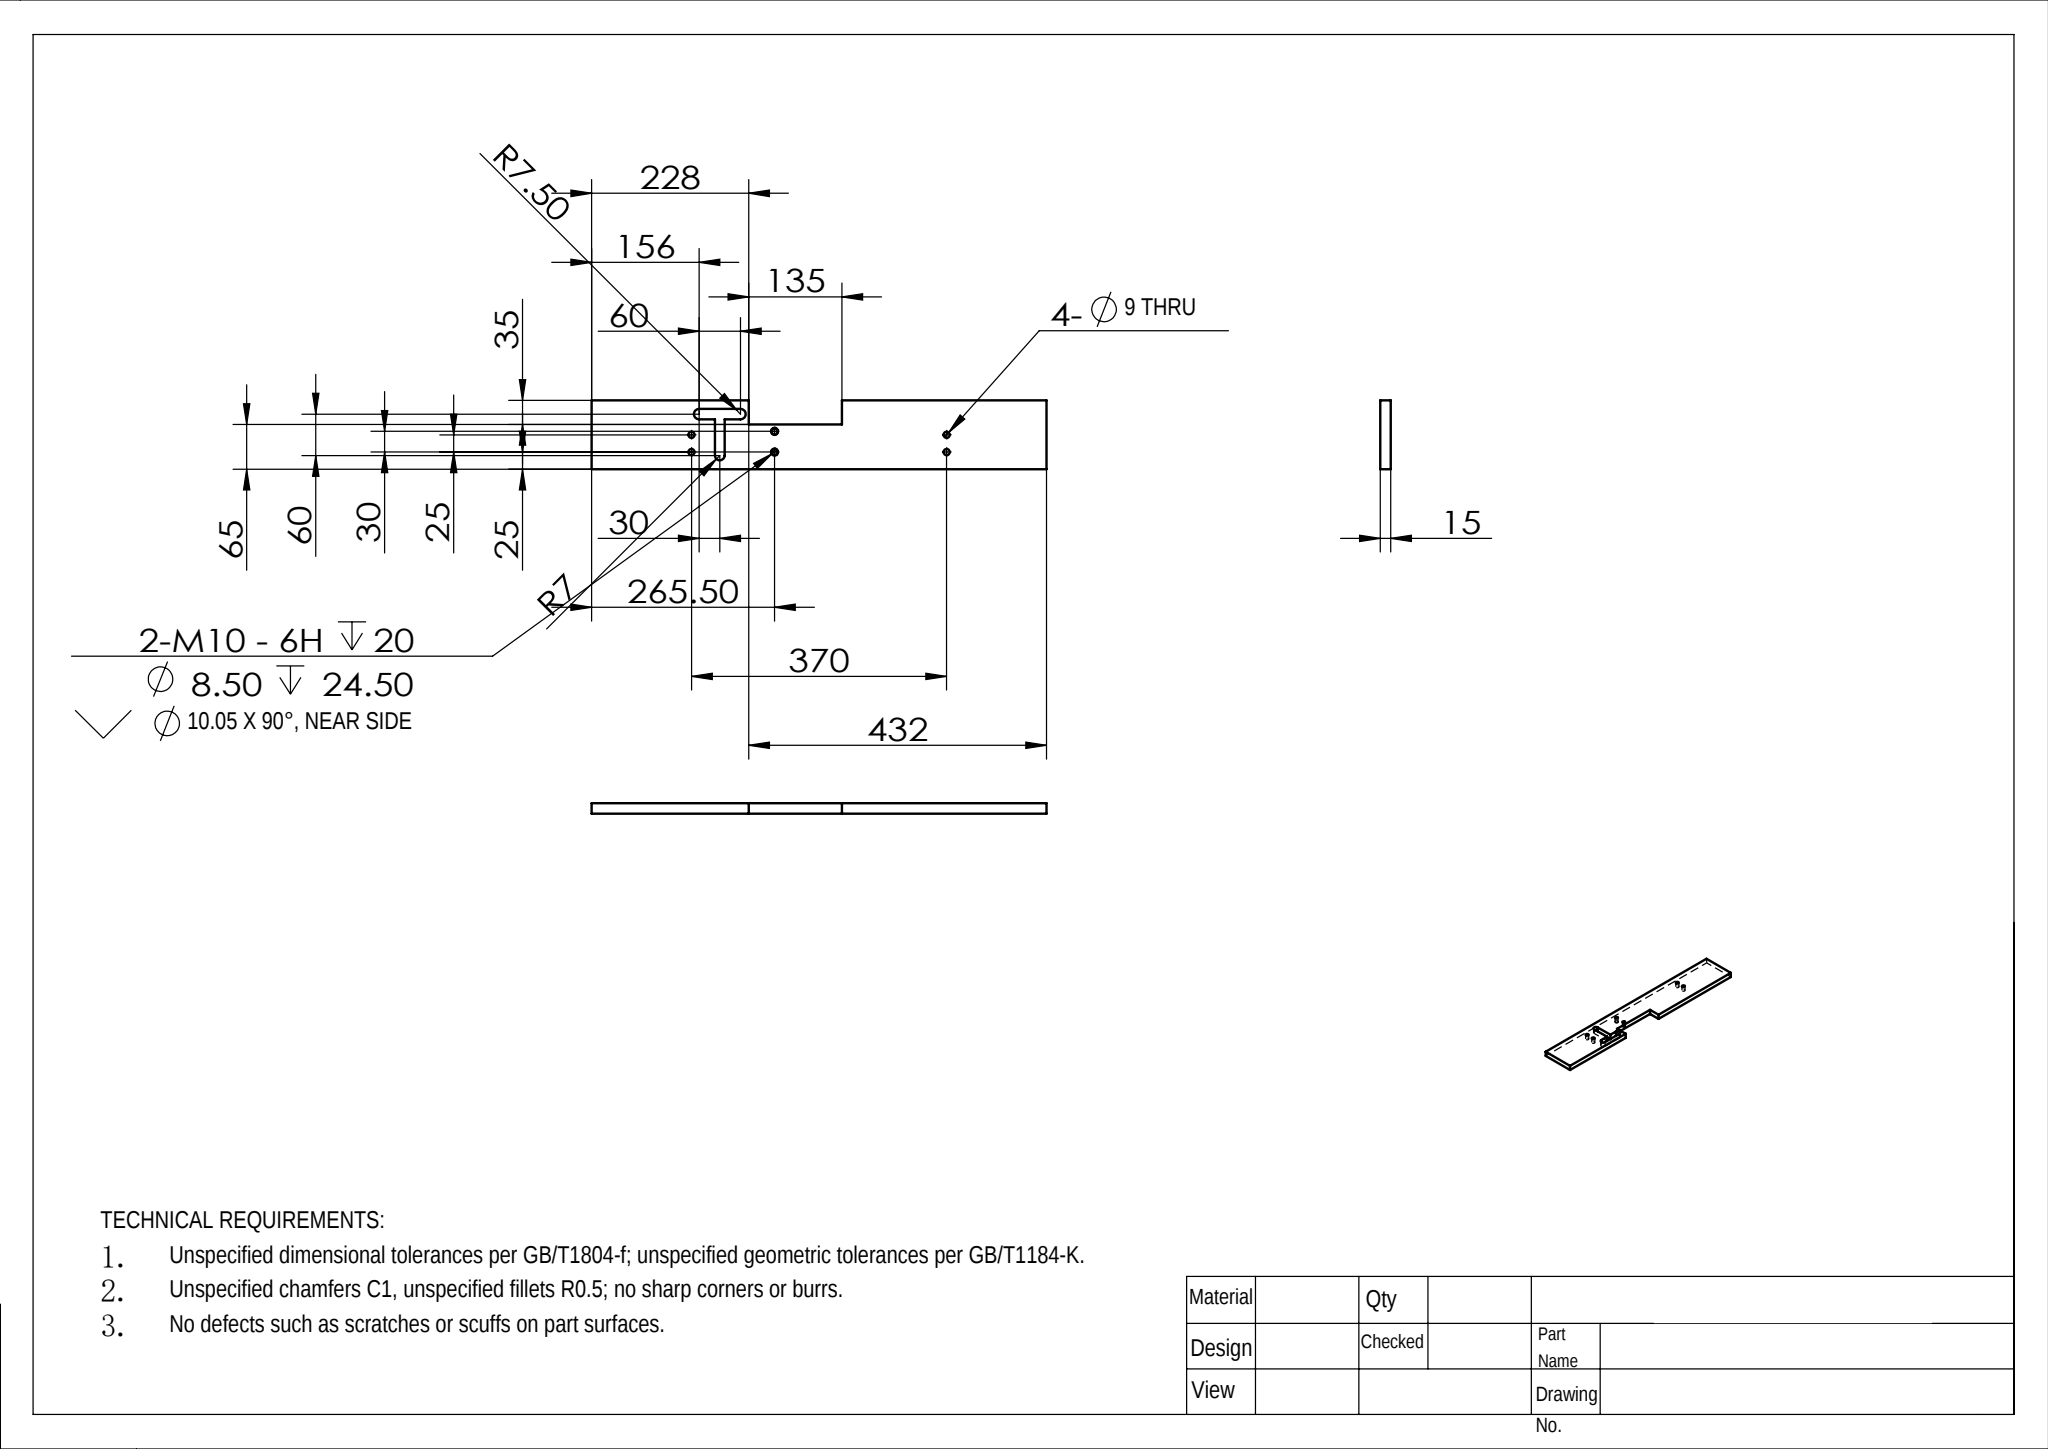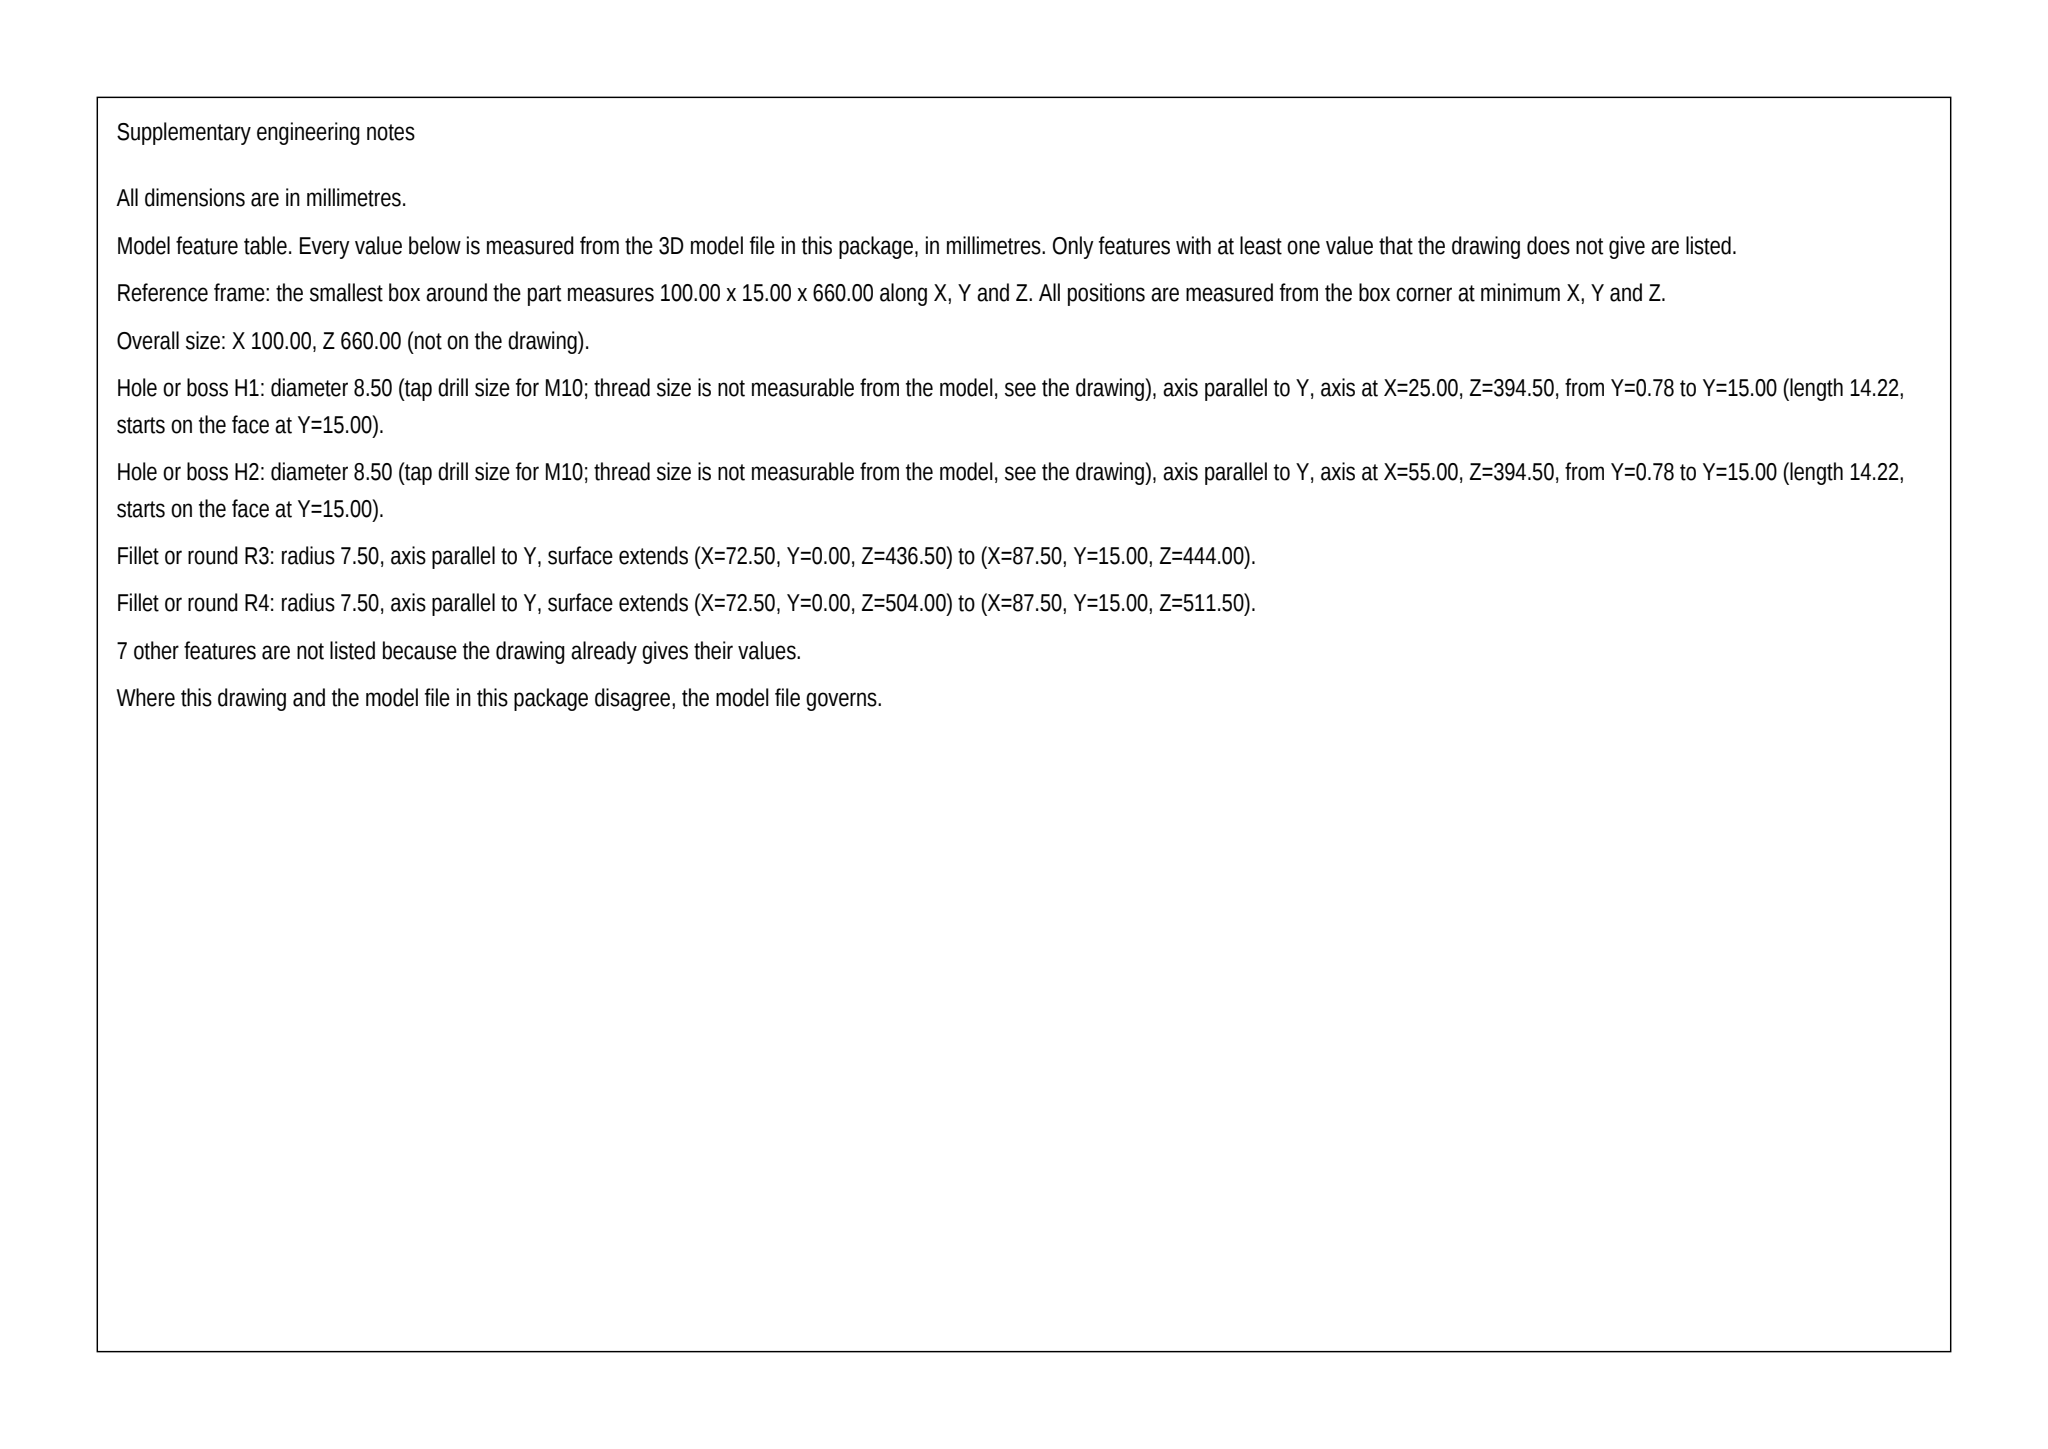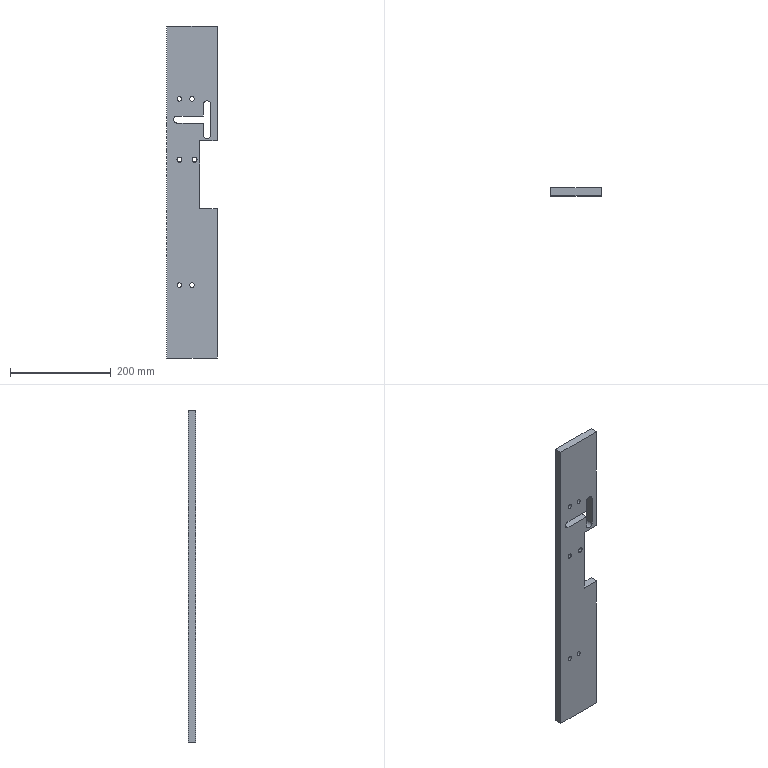Part | SolidWorks | mm | 1 solid | 35 faces | box 100 x 15 x 660 mm | volume 885258 mm3 | cylinder 16 | plane 15 | cone 4 | commonest cylinder face diameters 9 x8 8.5 x4 15 x3 14 x1
build123d program:
from build123d import *

# Parameters (mm, degrees)
SKETCH1_W                    = 100
SKETCH1_H                    = 660
BOSS_EXTRUDE1_DEPTH          = 15
M10_TAPPED_HOLE1_D           = 8.5
M10_TAPPED_HOLE1_DEPTH       = 24.5
M10_TAPPED_HOLE1_CSINK_D     = 10.05
M10_TAPPED_HOLE1_CSINK_ANGLE = 90
M10_TAPPED_HOLE1_TIP         = 2.554
SKETCH5_W                    = 66.431
SKETCH5_H                    = 135
CUT_EXTRUDE1_DEPTH           = 668.701
SKETCH6_R                    = 4.5
CUT_EXTRUDE2_DEPTH           = 668.701
CUT_EXTRUDE3_DEPTH           = 668.701
CUT_EXTRUDE4_DEPTH           = 668.701


with BuildPart() as part:
    # Sketch1 → Boss-Extrude1 (new body)
    with BuildSketch(Plane(origin=(0, 0, 0), x_dir=(1, 0, 0), z_dir=(0, 1, 0))):
        with Locations((50, 330)):
            Rectangle(SKETCH1_W, SKETCH1_H)
    extrude(amount=BOSS_EXTRUDE1_DEPTH)

    # M10 Tapped Hole1
    with Locations(Plane(origin=(0, 0, 0), x_dir=(-1, 0, 0), z_dir=(0, -1, 0))):
        with Locations((-55, 265.5), (-25, 265.5)):
            CounterSinkHole(M10_TAPPED_HOLE1_D / 2, M10_TAPPED_HOLE1_CSINK_D / 2, depth=M10_TAPPED_HOLE1_DEPTH, counter_sink_angle=M10_TAPPED_HOLE1_CSINK_ANGLE)
            with Locations((0, 0, -(M10_TAPPED_HOLE1_DEPTH + M10_TAPPED_HOLE1_TIP / 2))):  # 118° drill point
                Cone(0, M10_TAPPED_HOLE1_D / 2, M10_TAPPED_HOLE1_TIP, mode=Mode.SUBTRACT)

    # Sketch5 → Cut-Extrude1 (cut, through all)
    with BuildSketch(Plane(origin=(0, 15, 0), x_dir=(1, 0, 0), z_dir=(0, 1, 0))):
        with Locations((98.215, 295.5)):
            Rectangle(SKETCH5_W, SKETCH5_H)
    extrude(amount=-CUT_EXTRUDE1_DEPTH, mode=Mode.SUBTRACT)

    # Sketch6 → Cut-Extrude2 (cut, through all)
    with BuildSketch(Plane(origin=(0, 15, 0), x_dir=(1, 0, 0), z_dir=(0, 1, 0))):
        with Locations(Location((50, 515, 0), (0, 0, 270))):
            Circle(SKETCH6_R)
        with Locations(Location((25, 515, 0), (0, 0, 270))):
            Circle(SKETCH6_R)
        with Locations(Location((50, 145, 0), (0, 0, 270))):
            Circle(SKETCH6_R)
        with Locations(Location((25, 145, 0), (0, 0, 270))):
            Circle(SKETCH6_R)
    extrude(amount=-CUT_EXTRUDE2_DEPTH, mode=Mode.SUBTRACT)

    # Sketch7 → Cut-Extrude3 (cut, through all)
    with BuildSketch(Plane(origin=(0, 15, 0), x_dir=(1, 0, 0), z_dir=(0, 1, 0))):
        with BuildLine():
            Line((20, 193), (80, 193))
            ThreePointArc((80, 193), (87, 186), (80, 179))
            Line((80, 179), (20, 179))
            ThreePointArc((20, 179), (13, 186), (20, 193))
        make_face()
    extrude(amount=-CUT_EXTRUDE3_DEPTH, mode=Mode.SUBTRACT)

    # Sketch8 → Cut-Extrude4 (cut, through all)
    with BuildSketch(Plane(origin=(0, 15, 0), x_dir=(1, 0, 0), z_dir=(0, 1, 0))):
        with BuildLine():
            Line((72.5, 156), (72.5, 216))
            ThreePointArc((72.5, 216), (80, 223.5), (87.5, 216))
            Line((87.5, 216), (87.5, 156))
            ThreePointArc((87.5, 156), (80, 148.5), (72.5, 156))
        make_face()
    extrude(amount=-CUT_EXTRUDE4_DEPTH, mode=Mode.SUBTRACT)


solid = part.part